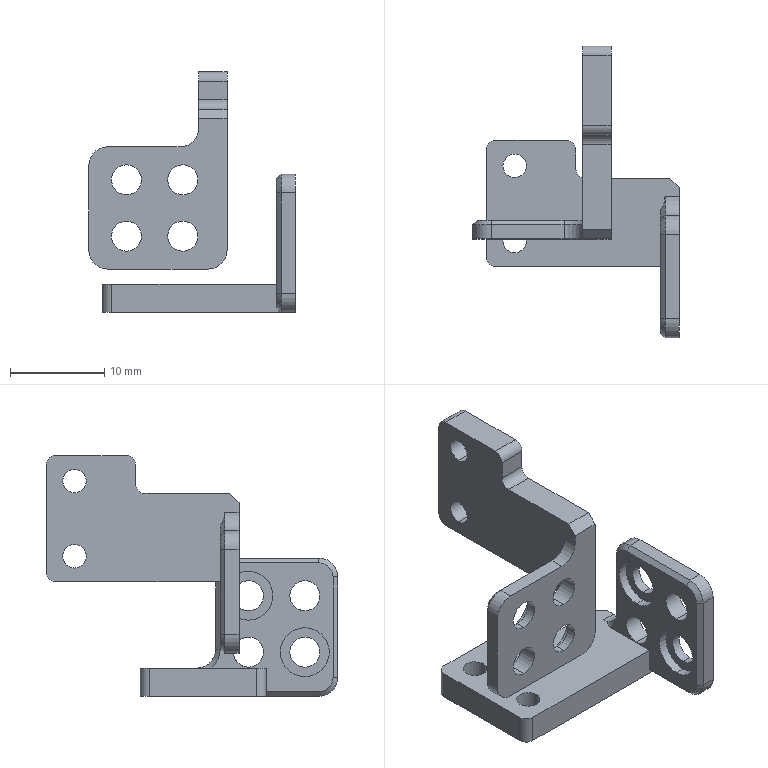CAM job | Mastercam | mm | 30 operations | part box 21.95 x 31 x 25.6
1. 3D High Speed (Area rest roughing) | 26 - 6 平铣刀
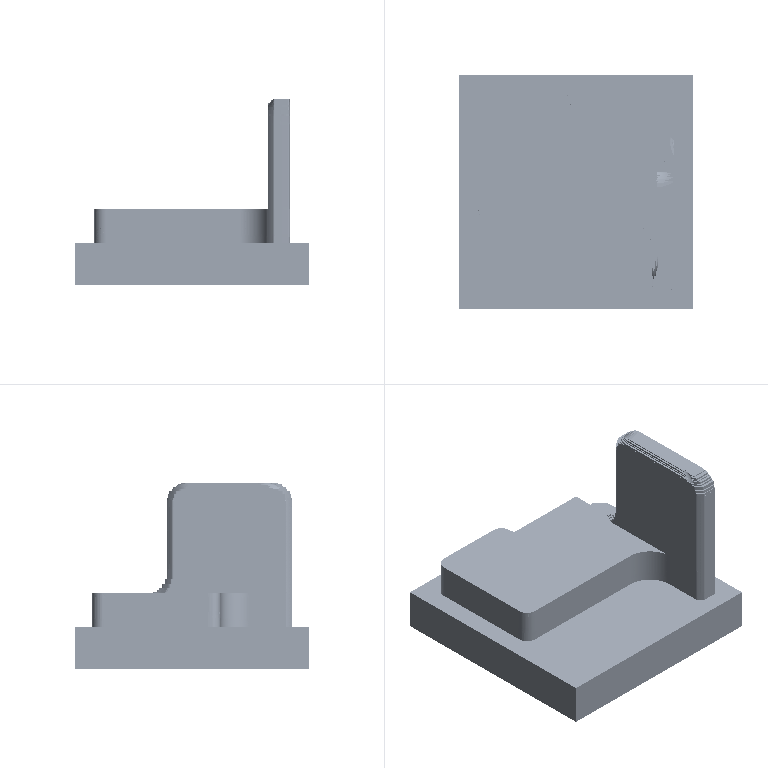2. 3D High Speed (Waterline rest passes) | 4 - 4C
3. Triangular mesh Triangular mesh | 5 - 4J
4. Contour (2D) | 5 - 4J
5. Contour (2D) | 5 - 4J
6. Contour (2D) | 5 - 4J
7. Drill/Counterbore | 6 - 6 倒角刀
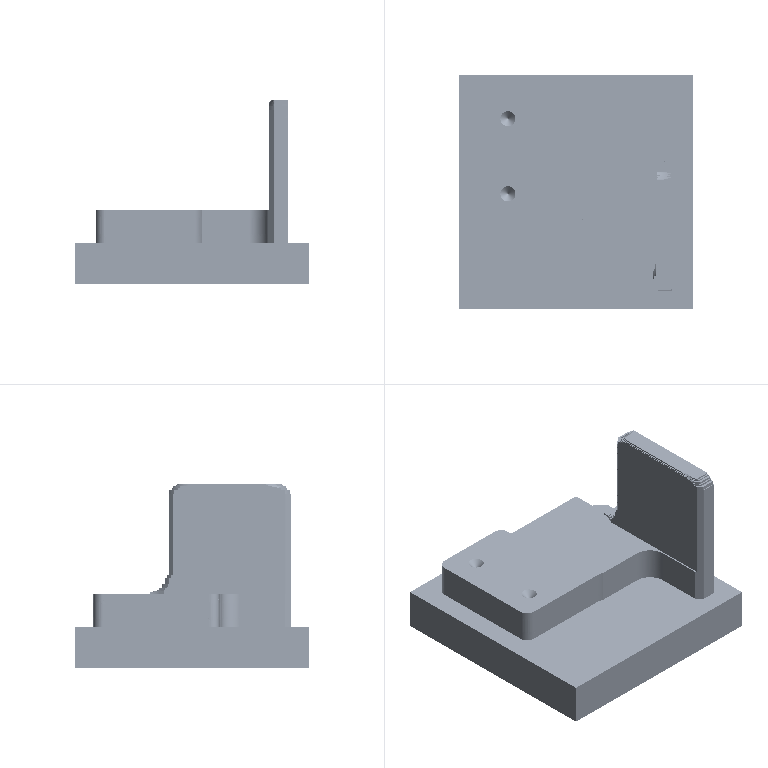8. Peck Drill | 8 - 2.5 钻头
9. Surface Finish Flowline | 15 - 4 圆鼻铣刀
10. Surface Finish Flowline | 15 - 4 圆鼻铣刀
11. Surface Finish Flowline | 15 - 4 圆鼻铣刀
12. Surface Finish Flowline | 15 - 4 圆鼻铣刀
13. Model Chamfer | 6 - 6 倒角刀
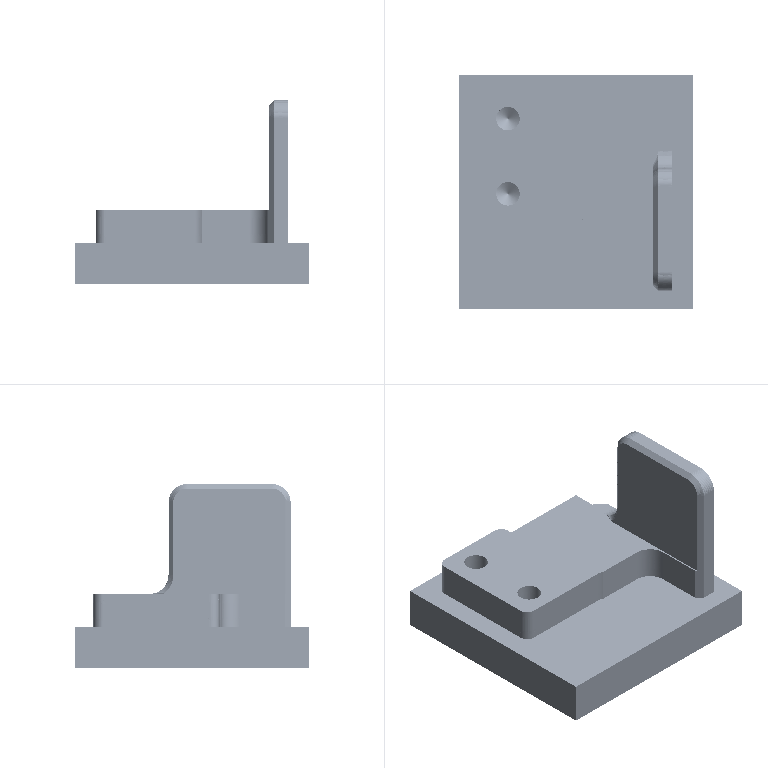14. Model Chamfer | 6 - 6 倒角刀
15. Chamfer Drill | 6 - 6 倒角刀
16. Model Chamfer | 6 - 6 倒角刀
17. Contour (Ramp) | 4 - 4C
18. Contour (2D) | 5 - 4J
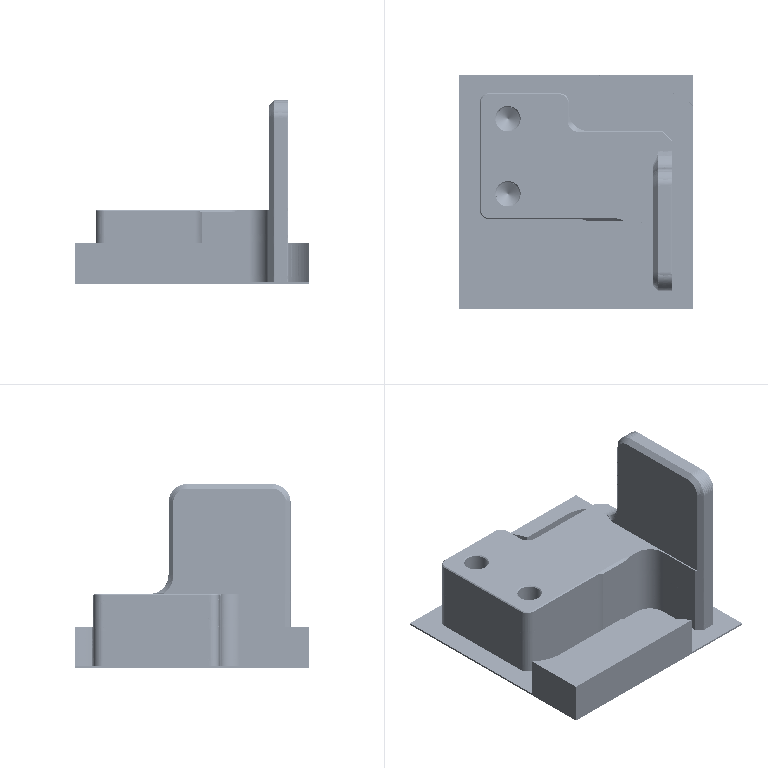19. Contour (Ramp) | 4 - 4C
20. Contour (2D) | 5 - 4J
21. Peck Drill | 10 - 3.2 钻头
22. Contour (Ramp) | 5 - 4J
23. Contour (2D) | 5 - 4J
24. Facing | 2 - 10C
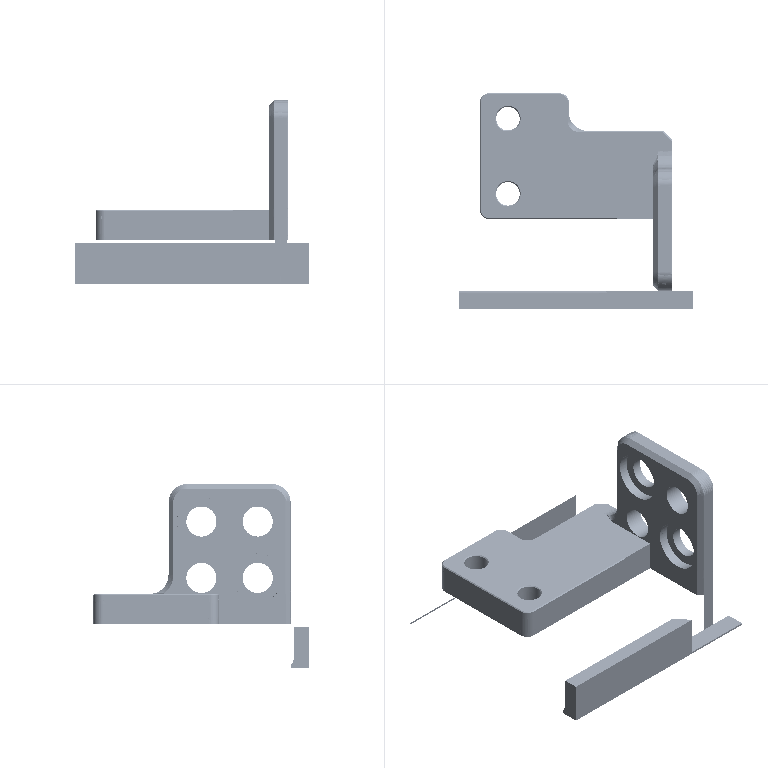25. Facing | 3 - 10J
26. Chamfer Drill | 11 - 4 倒角刀
27. Surface Finish Flowline | 15 - 4 圆鼻铣刀
28. 3D High Speed (Waterline) | 15 - 4 圆鼻铣刀
29. Contour (Remachining) | 13 - 2J
30. Model Chamfer | 11 - 4 倒角刀